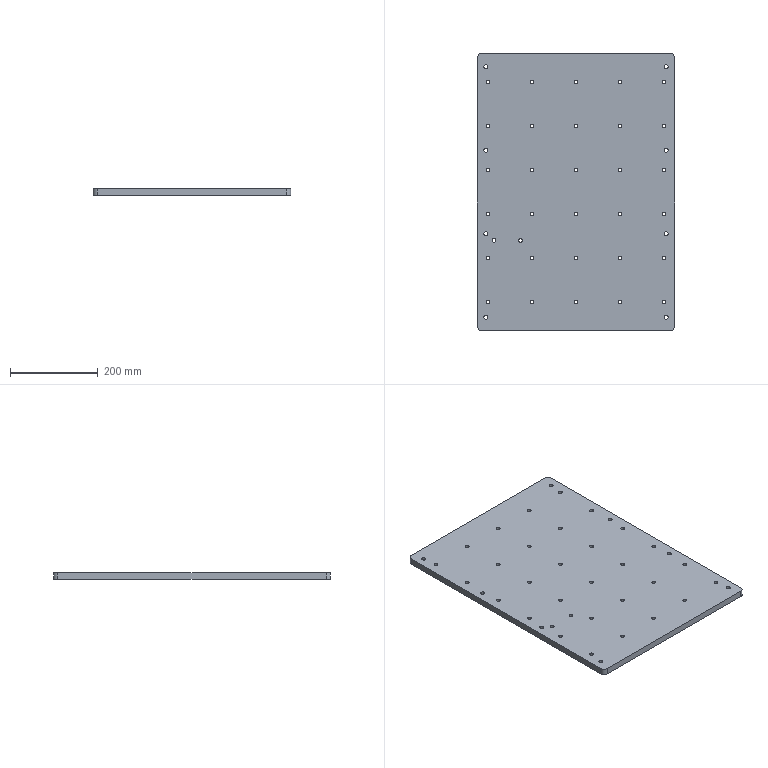CAM job | Mastercam | mm | 12 operations | part box 450 x 630 x 15
1. Contour (Ramp) | 16 - 16 平铣刀
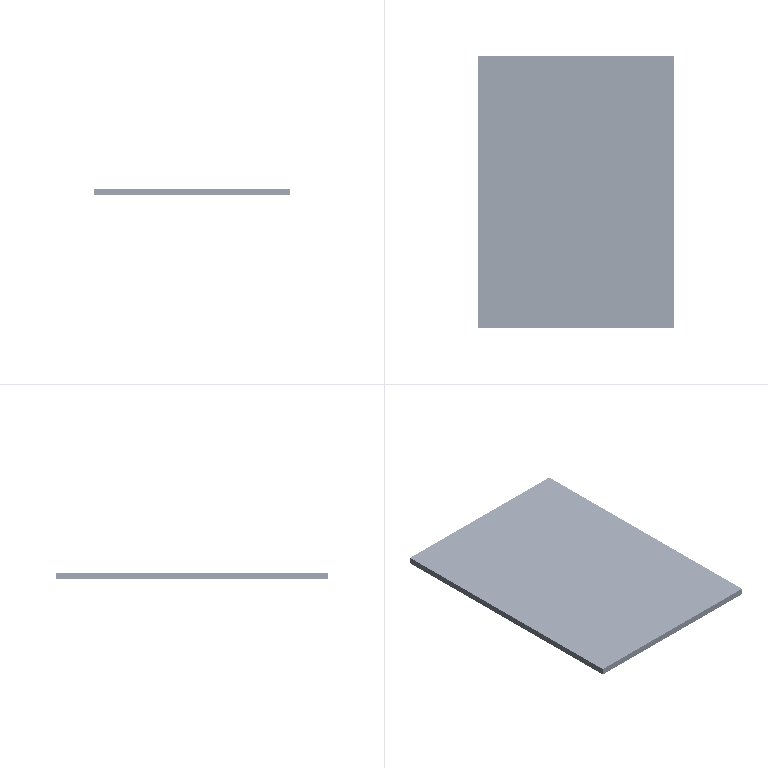2. Contour (2D) | 12 - 12 平铣刀
3. Contour (2D chamfer) | 7 - 4 倒角刀
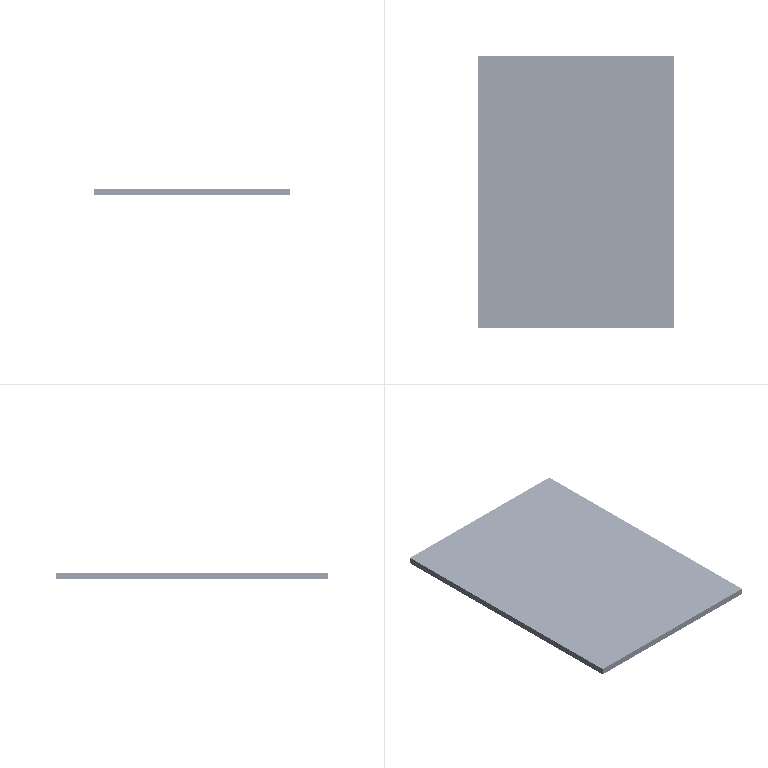4. Contour (Ramp) | 16 - 16 平铣刀
5. Contour (2D) | 12 - 12 平铣刀
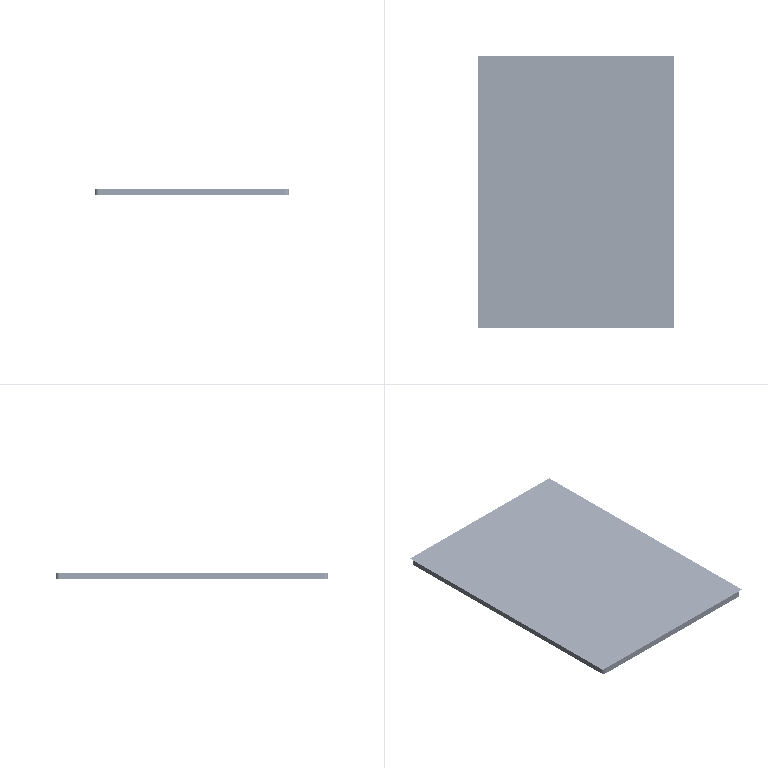6. Drill/Counterbore | 7 - 4 倒角刀
7. Peck Drill | 18 - 8.5 钻头
8. Contour (Ramp) | 8 - 8 平铣刀
9. Contour (2D) | 8 - 8 平铣刀
10. Contour (Ramp) | 5 - 5 平铣刀
11. Contour (2D) | 5 - 5 平铣刀
12. Contour (2D chamfer) | 7 - 4 倒角刀